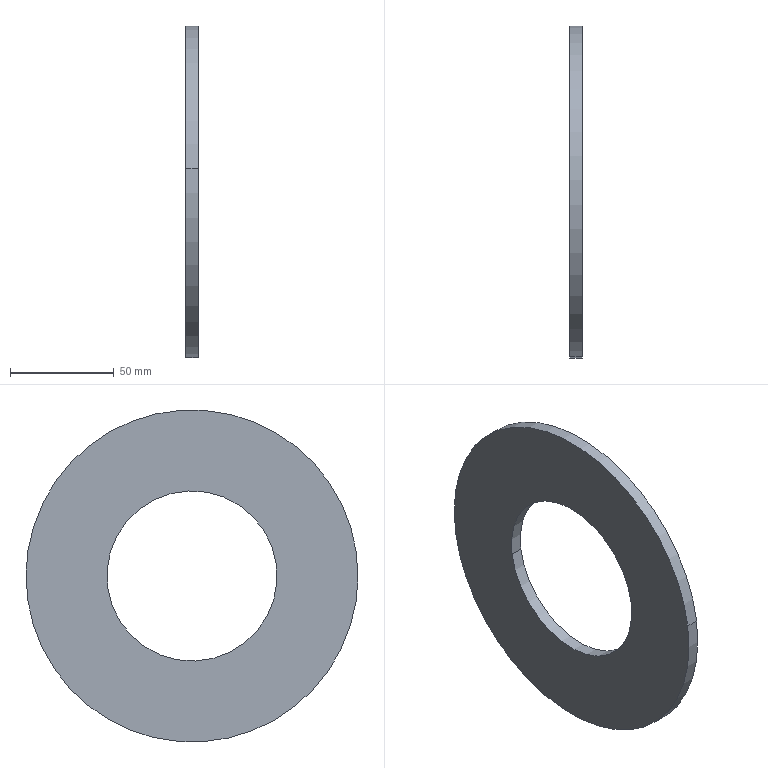Component | SolidWorks | Product-CopperFoilL587-2020-1 | 1 solid | 6 faces | box 6 x 160 x 160 mm | volume 88951 mm3 | cylinder 4 | plane 2 | commonest cylinder face diameters 82 x2 160 x2
build123d program:
from build123d import *

# Parameters (mm, degrees)
SKETCH1_R           = 80
SKETCH1_R_2         = 41
BOSS_EXTRUDE1_DEPTH = 6


with BuildPart() as part:
    # Sketch1 → Boss-Extrude1 (new body)
    with BuildSketch(Plane.XY):
        Circle(SKETCH1_R)
        Circle(SKETCH1_R_2, mode=Mode.SUBTRACT)
    extrude(amount=BOSS_EXTRUDE1_DEPTH)


solid = part.part

# Placed as in the assembly
solid = solid.moved(Location((2.716, -95.825, 207.018), (0, 90, 0)))
STEP:
#1=COLOUR_RGB('',0.7922,0.8196,0.9333);
#2=FILL_AREA_STYLE_COLOUR('',#1);
#3=FILL_AREA_STYLE('',(#2));
#4=SURFACE_STYLE_FILL_AREA(#3);
#5=SURFACE_SIDE_STYLE('',(#4));
#6=SURFACE_STYLE_USAGE(.BOTH.,#5);
#7=PRESENTATION_STYLE_ASSIGNMENT((#6));
#8=CARTESIAN_POINT('',(0.1069,-2.175,7.918));
#9=VERTEX_POINT('',#8);
#10=CARTESIAN_POINT('',(0.1069,-5.37,8.383));
#11=VERTEX_POINT('',#10);
#12=CARTESIAN_POINT('',(0.1069,-3.773,8.15));
#13=DIRECTION('',(-1.,-0.,0.));
#14=DIRECTION('',(0.,-0.9896,0.1441));
#15=AXIS2_PLACEMENT_3D('',#12,#13,#14);
#16=CIRCLE('',#15,1.614);
#17=EDGE_CURVE('',#9,#11,#16,.T.);
#18=ORIENTED_EDGE('',*,*,#17,.T.);
#19=CARTESIAN_POINT('',(0.3432,-5.37,8.383));
#20=VERTEX_POINT('',#19);
#21=CARTESIAN_POINT('',(0.1069,-5.37,8.383));
#22=DIRECTION('',(1.,0.,-0.));
#23=VECTOR('',#22,39.37);
#24=LINE('',#21,#23);
#25=EDGE_CURVE('',#11,#20,#24,.T.);
#26=ORIENTED_EDGE('',*,*,#25,.T.);
#27=CARTESIAN_POINT('',(0.3432,-2.175,7.918));
#28=VERTEX_POINT('',#27);
#29=CARTESIAN_POINT('',(0.3432,-3.773,8.15));
#30=DIRECTION('',(-1.,-0.,0.));
#31=DIRECTION('',(0.,-0.9896,0.1441));
#32=AXIS2_PLACEMENT_3D('',#29,#30,#31);
#33=CIRCLE('',#32,1.614);
#34=EDGE_CURVE('',#28,#20,#33,.T.);
#35=ORIENTED_EDGE('',*,*,#34,.F.);
#36=CARTESIAN_POINT('',(0.1069,-2.175,7.918));
#37=DIRECTION('',(1.,0.,-0.));
#38=VECTOR('',#37,39.37);
#39=LINE('',#36,#38);
#40=EDGE_CURVE('',#9,#28,#39,.T.);
#41=ORIENTED_EDGE('',*,*,#40,.F.);
#42=EDGE_LOOP('',(#18,#26,#35,#41));
#43=FACE_OUTER_BOUND('',#42,.T.);
#44=CARTESIAN_POINT('',(0.1069,-3.773,8.15));
#45=DIRECTION('',(1.,0.,-0.));
#46=DIRECTION('',(-0.,0.9896,-0.1441));
#47=AXIS2_PLACEMENT_3D('',#44,#45,#46);
#48=CYLINDRICAL_SURFACE('',#47,1.614);
#49=ADVANCED_FACE('',(#43),#48,.F.);
#50=CARTESIAN_POINT('',(0.1069,-6.889,8.604));
#51=VERTEX_POINT('',#50);
#52=CARTESIAN_POINT('',(0.1069,-0.6559,7.697));
#53=VERTEX_POINT('',#52);
#54=CARTESIAN_POINT('',(0.1069,-3.773,8.15));
#55=DIRECTION('',(-1.,-0.,0.));
#56=DIRECTION('',(0.,-0.9896,0.1441));
#57=AXIS2_PLACEMENT_3D('',#54,#55,#56);
#58=CIRCLE('',#57,3.15);
#59=EDGE_CURVE('',#51,#53,#58,.T.);
#60=ORIENTED_EDGE('',*,*,#59,.F.);
#61=CARTESIAN_POINT('',(0.3432,-6.889,8.604));
#62=VERTEX_POINT('',#61);
#63=CARTESIAN_POINT('',(0.1069,-6.889,8.604));
#64=DIRECTION('',(1.,0.,-0.));
#65=VECTOR('',#64,39.37);
#66=LINE('',#63,#65);
#67=EDGE_CURVE('',#51,#62,#66,.T.);
#68=ORIENTED_EDGE('',*,*,#67,.T.);
#69=CARTESIAN_POINT('',(0.3432,-0.6559,7.697));
#70=VERTEX_POINT('',#69);
#71=CARTESIAN_POINT('',(0.3432,-3.773,8.15));
#72=DIRECTION('',(-1.,-0.,0.));
#73=DIRECTION('',(0.,-0.9896,0.1441));
#74=AXIS2_PLACEMENT_3D('',#71,#72,#73);
#75=CIRCLE('',#74,3.15);
#76=EDGE_CURVE('',#62,#70,#75,.T.);
#77=ORIENTED_EDGE('',*,*,#76,.T.);
#78=CARTESIAN_POINT('',(0.1069,-0.6559,7.697));
#79=DIRECTION('',(1.,0.,-0.));
#80=VECTOR('',#79,39.37);
#81=LINE('',#78,#80);
#82=EDGE_CURVE('',#53,#70,#81,.T.);
#83=ORIENTED_EDGE('',*,*,#82,.F.);
#84=EDGE_LOOP('',(#60,#68,#77,#83));
#85=FACE_OUTER_BOUND('',#84,.T.);
#86=CARTESIAN_POINT('',(0.1069,-3.773,8.15));
#87=DIRECTION('',(1.,0.,-0.));
#88=DIRECTION('',(-0.,0.9896,-0.1441));
#89=AXIS2_PLACEMENT_3D('',#86,#87,#88);
#90=CYLINDRICAL_SURFACE('',#89,3.15);
#91=ADVANCED_FACE('',(#85),#90,.T.);
#92=CARTESIAN_POINT('',(0.1069,-3.773,8.15));
#93=DIRECTION('',(-1.,-0.,0.));
#94=DIRECTION('',(0.,-0.9896,0.1441));
#95=AXIS2_PLACEMENT_3D('',#92,#93,#94);
#96=CIRCLE('',#95,3.15);
#97=EDGE_CURVE('',#53,#51,#96,.T.);
#98=ORIENTED_EDGE('',*,*,#97,.T.);
#99=ORIENTED_EDGE('',*,*,#59,.T.);
#100=EDGE_LOOP('',(#98,#99));
#101=FACE_OUTER_BOUND('',#100,.T.);
#102=ORIENTED_EDGE('',*,*,#17,.F.);
#103=CARTESIAN_POINT('',(0.1069,-3.773,8.15));
#104=DIRECTION('',(-1.,-0.,0.));
#105=DIRECTION('',(0.,-0.9896,0.1441));
#106=AXIS2_PLACEMENT_3D('',#103,#104,#105);
#107=CIRCLE('',#106,1.614);
#108=EDGE_CURVE('',#11,#9,#107,.T.);
#109=ORIENTED_EDGE('',*,*,#108,.F.);
#110=EDGE_LOOP('',(#102,#109));
#111=FACE_BOUND('',#110,.T.);
#112=CARTESIAN_POINT('',(0.1069,-3.773,8.15));
#113=DIRECTION('',(-1.,-0.,0.));
#114=DIRECTION('',(0.,-0.9896,0.1441));
#115=AXIS2_PLACEMENT_3D('',#112,#113,#114);
#116=PLANE('',#115);
#117=ADVANCED_FACE('',(#101,#111),#116,.T.);
#118=CARTESIAN_POINT('',(0.3432,-3.773,8.15));
#119=DIRECTION('',(-1.,-0.,0.));
#120=DIRECTION('',(0.,-0.9896,0.1441));
#121=AXIS2_PLACEMENT_3D('',#118,#119,#120);
#122=CIRCLE('',#121,3.15);
#123=EDGE_CURVE('',#70,#62,#122,.T.);
#124=ORIENTED_EDGE('',*,*,#123,.F.);
#125=ORIENTED_EDGE('',*,*,#76,.F.);
#126=EDGE_LOOP('',(#124,#125));
#127=FACE_OUTER_BOUND('',#126,.T.);
#128=ORIENTED_EDGE('',*,*,#34,.T.);
#129=CARTESIAN_POINT('',(0.3432,-3.773,8.15));
#130=DIRECTION('',(-1.,-0.,0.));
#131=DIRECTION('',(0.,-0.9896,0.1441));
#132=AXIS2_PLACEMENT_3D('',#129,#130,#131);
#133=CIRCLE('',#132,1.614);
#134=EDGE_CURVE('',#20,#28,#133,.T.);
#135=ORIENTED_EDGE('',*,*,#134,.T.);
#136=EDGE_LOOP('',(#128,#135));
#137=FACE_BOUND('',#136,.T.);
#138=CARTESIAN_POINT('',(0.3432,-3.773,8.15));
#139=DIRECTION('',(-1.,-0.,0.));
#140=DIRECTION('',(0.,-0.9896,0.1441));
#141=AXIS2_PLACEMENT_3D('',#138,#139,#140);
#142=PLANE('',#141);
#143=ADVANCED_FACE('',(#127,#137),#142,.F.);
#144=ORIENTED_EDGE('',*,*,#67,.F.);
#145=ORIENTED_EDGE('',*,*,#97,.F.);
#146=ORIENTED_EDGE('',*,*,#82,.T.);
#147=ORIENTED_EDGE('',*,*,#123,.T.);
#148=EDGE_LOOP('',(#144,#145,#146,#147));
#149=FACE_OUTER_BOUND('',#148,.T.);
#150=CARTESIAN_POINT('',(0.1069,-3.773,8.15));
#151=DIRECTION('',(1.,0.,-0.));
#152=DIRECTION('',(-0.,0.9896,-0.1441));
#153=AXIS2_PLACEMENT_3D('',#150,#151,#152);
#154=CYLINDRICAL_SURFACE('',#153,3.15);
#155=ADVANCED_FACE('',(#149),#154,.T.);
#156=ORIENTED_EDGE('',*,*,#25,.F.);
#157=ORIENTED_EDGE('',*,*,#108,.T.);
#158=ORIENTED_EDGE('',*,*,#40,.T.);
#159=ORIENTED_EDGE('',*,*,#134,.F.);
#160=EDGE_LOOP('',(#156,#157,#158,#159));
#161=FACE_OUTER_BOUND('',#160,.T.);
#162=CARTESIAN_POINT('',(0.1069,-3.773,8.15));
#163=DIRECTION('',(1.,0.,-0.));
#164=DIRECTION('',(-0.,0.9896,-0.1441));
#165=AXIS2_PLACEMENT_3D('',#162,#163,#164);
#166=CYLINDRICAL_SURFACE('',#165,1.614);
#167=ADVANCED_FACE('',(#161),#166,.F.);
#168=CLOSED_SHELL('',(#49,#91,#117,#143,#155,#167));
#169=MANIFOLD_SOLID_BREP('',#168);
#170=STYLED_ITEM('',(#7),#169);
#171=PRESENTATION_LAYER_ASSIGNMENT('','',(#170));
#172=CARTESIAN_POINT('',(0.,0.,0.));
#173=DIRECTION('',(0.,0.,1.));
#174=DIRECTION('',(1.,0.,0.));
#175=AXIS2_PLACEMENT_3D('',#172,#173,#174);
#176=(LENGTH_UNIT()NAMED_UNIT(*)SI_UNIT($,.METRE.));
#177=LENGTH_MEASURE_WITH_UNIT(LENGTH_MEASURE(0.0254),#176);
#178=DIMENSIONAL_EXPONENTS(1.,0.,0.,0.,0.,0.,0.);
#179=(CONVERSION_BASED_UNIT('',#177)LENGTH_UNIT()NAMED_UNIT(#178));
#180=UNCERTAINTY_MEASURE_WITH_UNIT(LENGTH_MEASURE(0.00001),#179,'','');
#181=(NAMED_UNIT(*)PLANE_ANGLE_UNIT()SI_UNIT($,.RADIAN.));
#182=(NAMED_UNIT(*)SI_UNIT($,.STERADIAN.)SOLID_ANGLE_UNIT());
#183=(GEOMETRIC_REPRESENTATION_CONTEXT(3)GLOBAL_UNCERTAINTY_ASSIGNED_CONTEXT((#180))GLOBAL_UNIT_ASSIGNED_CONTEXT((#179,#181,#182))REPRESENTATION_CONTEXT('',''));
#184=ADVANCED_BREP_SHAPE_REPRESENTATION('',(#169,#175),#183);
#185=(LENGTH_UNIT()NAMED_UNIT(*)SI_UNIT($,.METRE.));
#186=LENGTH_MEASURE_WITH_UNIT(LENGTH_MEASURE(0.0254),#185);
#187=DIMENSIONAL_EXPONENTS(1.,0.,0.,0.,0.,0.,0.);
#188=(CONVERSION_BASED_UNIT('',#186)LENGTH_UNIT()NAMED_UNIT(#187));
#189=UNCERTAINTY_MEASURE_WITH_UNIT(LENGTH_MEASURE(0.00001),#188,'','');
#190=(NAMED_UNIT(*)PLANE_ANGLE_UNIT()SI_UNIT($,.RADIAN.));
#191=(NAMED_UNIT(*)SI_UNIT($,.STERADIAN.)SOLID_ANGLE_UNIT());
#192=(GEOMETRIC_REPRESENTATION_CONTEXT(3)GLOBAL_UNCERTAINTY_ASSIGNED_CONTEXT((#189))GLOBAL_UNIT_ASSIGNED_CONTEXT((#188,#190,#191))REPRESENTATION_CONTEXT('',''));
#193=MECHANICAL_DESIGN_GEOMETRIC_PRESENTATION_REPRESENTATION('',(#170),#192);